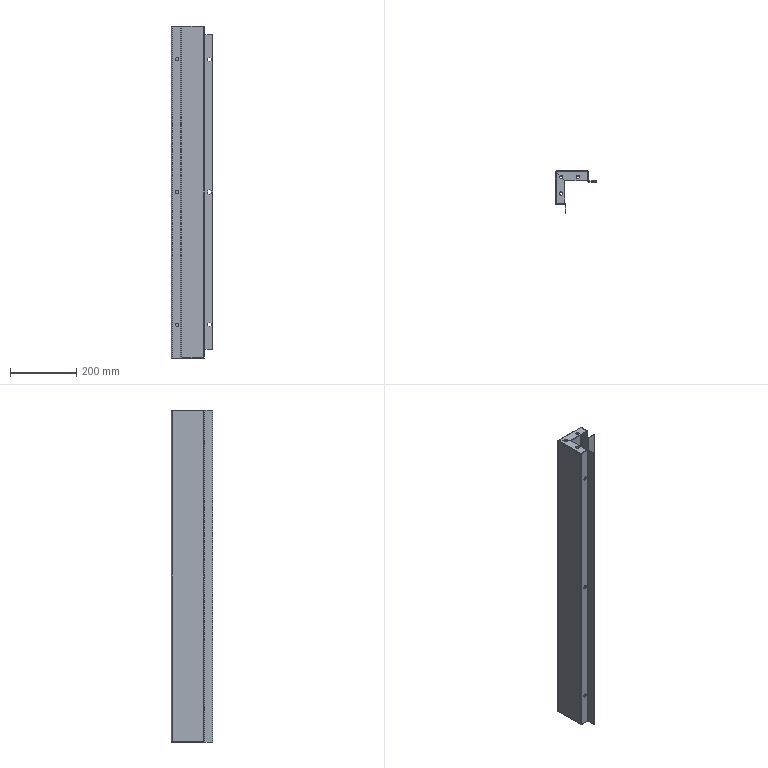Component | SolidWorks | 15UpperLeftBeam-1 | 1 solid | 126 faces | volume 618891 mm3 | plane 84 | cylinder 38 | spline 4 | commonest cylinder face diameters 10 x20 6 x9 2 x9